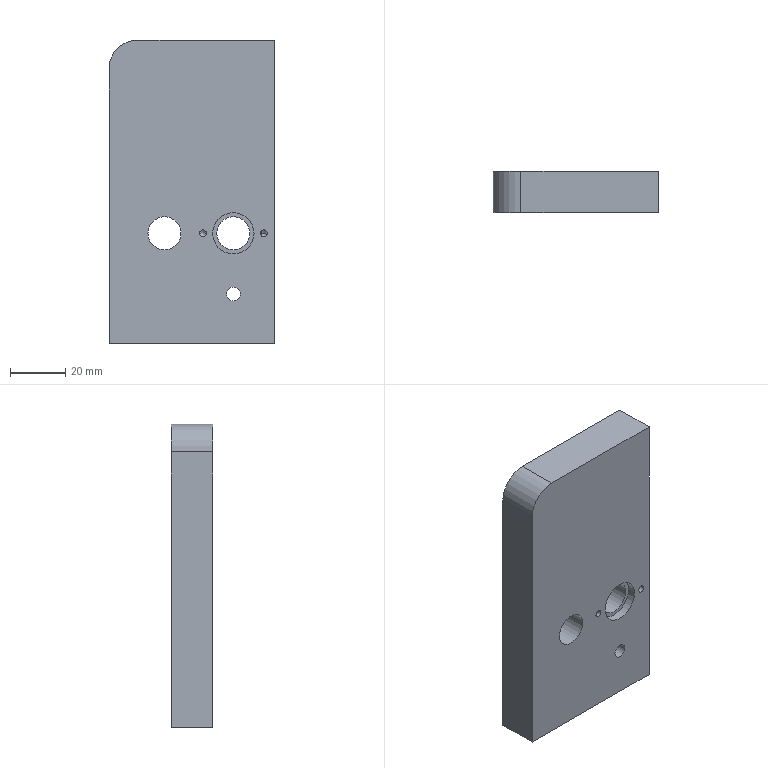Component | SolidWorks | GbgbSupportPlateF8-1 | 1 solid | 65 faces | box 60 x 15 x 110 mm | volume 88746 mm3 | cylinder 34 | cone 18 | plane 13 | commonest cylinder face diameters 3.3 x10 2.5 x8 6 x4 12 x4 4 x3 5 x2 15 x2 20 x1
build123d program:
from build123d import *

# Parameters (mm, degrees)
SKETCH1_W             = 60
SKETCH1_H             = 110
BOSS_EXTRUDE1_DEPTH   = 15
SKETCH2_W             = 20
SKETCH2_H             = 80
CUT_EXTRUDE1_DEPTH    = 3.1
SKETCH3_R             = 6
SKETCH3_R_2           = 1
CUT_EXTRUDE2_DEPTH    = 64.77
M4_TAPPED_HOLE1_D     = 3.3
M4_TAPPED_HOLE1_DEPTH = 10.1
M4_TAPPED_HOLE1_TIP   = 0.9914
SKETCH6_R             = 6
CUT_EXTRUDE3_DEPTH    = 65.42
M3_TAPPED_HOLE1_D     = 2.5
M3_TAPPED_HOLE1_DEPTH = 7.5
M3_TAPPED_HOLE1_TIP   = 0.7511
M4_TAPPED_HOLE3_D     = 3.3
M4_TAPPED_HOLE3_DEPTH = 10.1
M4_TAPPED_HOLE3_TIP   = 0.9914
FILLET1_R             = 10
SKETCH14_R            = 7.5
CUT_EXTRUDE5_DEPTH    = 3
SKETCH15_R            = 3
CUT_EXTRUDE6_DEPTH    = 15
SKETCH16_R            = 2
CUT_EXTRUDE7_DEPTH    = 3.1
M6_TAPPED_HOLE1_D     = 5
M6_TAPPED_HOLE1_DEPTH = 15
M6_TAPPED_HOLE1_TIP   = 1.502
M3_TAPPED_HOLE2_D     = 2.5
M3_TAPPED_HOLE2_DEPTH = 7.5
M3_TAPPED_HOLE2_TIP   = 0.7511


with BuildPart() as part:
    # Sketch1 → Boss-Extrude1 (new body)
    with BuildSketch(Plane.XY):
        Rectangle(SKETCH1_W, SKETCH1_H)
    extrude(amount=BOSS_EXTRUDE1_DEPTH)

    # Sketch2 → Cut-Extrude1 (cut)
    with BuildSketch(Plane.XY.offset(15)):
        with Locations((15, 15)):
            Rectangle(SKETCH2_W, SKETCH2_H)
    extrude(amount=-CUT_EXTRUDE1_DEPTH, mode=Mode.SUBTRACT)

    # Sketch3 → Cut-Extrude2 (cut, through all)
    with BuildSketch(Plane.XY.offset(11.9)):
        with Locations((15, 15)):
            Circle(SKETCH3_R)
        with Locations((15, 37)):
            Circle(SKETCH3_R_2)
    extrude(amount=-CUT_EXTRUDE2_DEPTH, mode=Mode.SUBTRACT)

    # M4 Tapped Hole1
    with Locations(Plane(origin=(0, 55, 0), x_dir=(1, 0, 0), z_dir=(0, 1, 0))):
        with Locations((25, -5), (0, -5), (-25, -5)):
            Hole(M4_TAPPED_HOLE1_D / 2, depth=M4_TAPPED_HOLE1_DEPTH)
            with Locations((0, 0, -(M4_TAPPED_HOLE1_DEPTH + M4_TAPPED_HOLE1_TIP / 2))):  # 118° drill point
                Cone(0, M4_TAPPED_HOLE1_D / 2, M4_TAPPED_HOLE1_TIP, mode=Mode.SUBTRACT)

    # Sketch6 → Cut-Extrude3 (cut, through all)
    with BuildSketch(Plane.XY.offset(15)):
        with Locations((-10, 15)):
            Circle(SKETCH6_R)
    extrude(amount=-CUT_EXTRUDE3_DEPTH, mode=Mode.SUBTRACT)

    # M3 Tapped Hole1
    with Locations(Plane(origin=(0, 0, 0), x_dir=(-1, 0, 0), z_dir=(0, 0, -1))):
        with Locations((-26, 15), (-4, 15)):
            Hole(M3_TAPPED_HOLE1_D / 2, depth=M3_TAPPED_HOLE1_DEPTH)
            with Locations((0, 0, -(M3_TAPPED_HOLE1_DEPTH + M3_TAPPED_HOLE1_TIP / 2))):  # 118° drill point
                Cone(0, M3_TAPPED_HOLE1_D / 2, M3_TAPPED_HOLE1_TIP, mode=Mode.SUBTRACT)

    # M4 Tapped Hole3
    with Locations(Plane.XY.offset(15)):
        with Locations((-20, 22.5), (-20, 7.5)):
            Hole(M4_TAPPED_HOLE3_D / 2, depth=M4_TAPPED_HOLE3_DEPTH)
            with Locations((0, 0, -(M4_TAPPED_HOLE3_DEPTH + M4_TAPPED_HOLE3_TIP / 2))):  # 118° drill point
                Cone(0, M4_TAPPED_HOLE3_D / 2, M4_TAPPED_HOLE3_TIP, mode=Mode.SUBTRACT)

    # Fillet1
    fillet1_edges = [part.edges().sort_by_distance(p)[0] for p in [
        (-30, -55, 7.5),
    ]]
    fillet(fillet1_edges, radius=FILLET1_R)

    # Sketch14 → Cut-Extrude5 (cut)
    with BuildSketch(Plane(origin=(0, 0, 0), x_dir=(-1, 0, 0), z_dir=(0, 0, -1))):
        with Locations((-15, 15)):
            Circle(SKETCH14_R)
    extrude(amount=-CUT_EXTRUDE5_DEPTH, mode=Mode.SUBTRACT)

    # Sketch15 → Cut-Extrude6 (cut)
    with BuildSketch(Plane(origin=(0, 55, 0), x_dir=(1, 0, 0), z_dir=(0, 1, 0))):
        with Locations(Location((-15, -5, 0), (0, 0, 270))):
            Circle(SKETCH15_R)
        with Locations(Location((15, -5, 0), (0, 0, 270))):
            Circle(SKETCH15_R)
    extrude(amount=-CUT_EXTRUDE6_DEPTH, mode=Mode.SUBTRACT)

    # Sketch16 → Cut-Extrude7 (cut)
    with BuildSketch(Plane.XY.offset(15)):
        with Locations((5, -25)):
            Circle(SKETCH16_R)
        with Locations((25, -25)):
            Circle(SKETCH16_R)
    extrude(amount=-CUT_EXTRUDE7_DEPTH, mode=Mode.SUBTRACT)

    # M6 Tapped Hole1
    with Locations(Plane.XY.offset(11.9)):
        with Locations((15, 37)):
            Hole(M6_TAPPED_HOLE1_D / 2, depth=M6_TAPPED_HOLE1_DEPTH)
            with Locations((0, 0, -(M6_TAPPED_HOLE1_DEPTH + M6_TAPPED_HOLE1_TIP / 2))):  # 118° drill point
                Cone(0, M6_TAPPED_HOLE1_D / 2, M6_TAPPED_HOLE1_TIP, mode=Mode.SUBTRACT)

    # M3 Tapped Hole2
    with Locations(Plane.XY.offset(15)):
        with Locations((9.5, -46), (20.5, -46)):
            Hole(M3_TAPPED_HOLE2_D / 2, depth=M3_TAPPED_HOLE2_DEPTH)
            with Locations((0, 0, -(M3_TAPPED_HOLE2_DEPTH + M3_TAPPED_HOLE2_TIP / 2))):  # 118° drill point
                Cone(0, M3_TAPPED_HOLE2_D / 2, M3_TAPPED_HOLE2_TIP, mode=Mode.SUBTRACT)


solid = part.part

# Placed as in the assembly
solid = solid.moved(Location((65.446, 372.44, 445.232), (-90, 0, 0)))